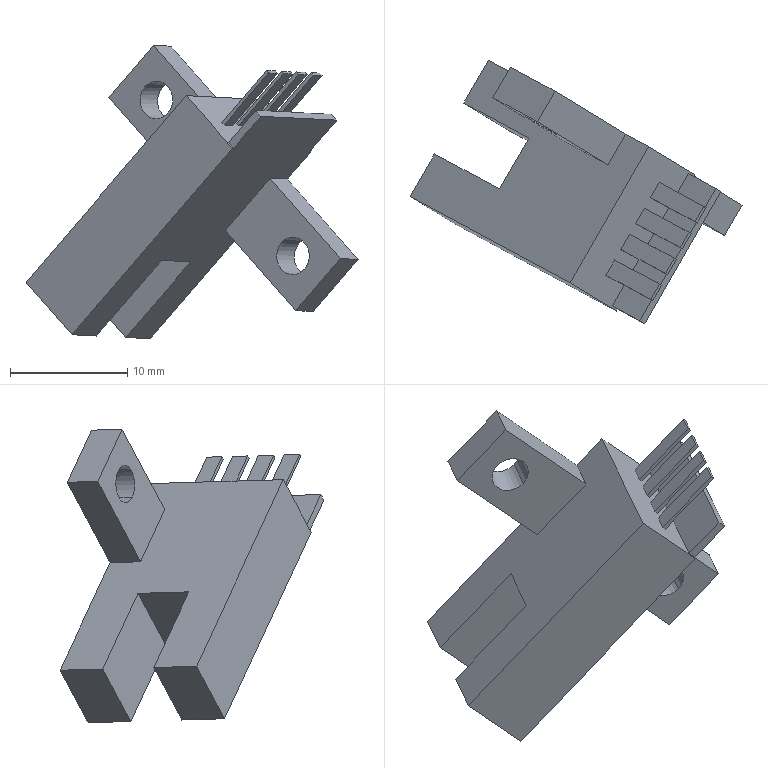Component | SolidWorks | KKSwitch-0710z0-123-1_EE-SX672-0710z0-123-4 | 1 solid | 46 faces | box 28.26 x 22.46 x 24.98 mm | volume 1978 mm3 | plane 42 | cylinder 4 | commonest cylinder face diameters 3.2 x4
build123d program:
from build123d import *

# Parameters (mm, degrees)
SKETCH1_W           = 13.4
SKETCH1_H           = 22.2
BOSS_EXTRUDE1_DEPTH = 6.4
SKETCH2_W           = 5
SKETCH2_H           = 9
CUT_EXTRUDE1_DEPTH  = 27.709
SKETCH3_W           = 1.5
SKETCH3_H           = 0.3
BOSS_EXTRUDE2_DEPTH = 6.2
SKETCH4_W           = 1.5
SKETCH4_H           = 0.3
BOSS_EXTRUDE3_DEPTH = 6.2
SKETCH5_W           = 1.5
SKETCH5_H           = 0.3
BOSS_EXTRUDE4_DEPTH = 6.2
SKETCH6_W           = 3
SKETCH6_H           = 6.2
BOSS_EXTRUDE5_DEPTH = 9.8
SKETCH7_W           = 3
SKETCH7_H           = 6.2
BOSS_EXTRUDE6_DEPTH = 9.8
SKETCH8_W           = 13
SKETCH8_H           = 0.7
BOSS_EXTRUDE7_DEPTH = 3.8
SKETCH9_W           = 1.5
SKETCH9_H           = 0.3
BOSS_EXTRUDE8_DEPTH = 6.2
DRILL1_D            = 3.2
DRILL2_D            = 3.2


with BuildPart() as part:
    # Sketch1 → Boss-Extrude1 (new body)
    with BuildSketch(Plane(origin=(0, 0, 0), x_dir=(-1, 0, 0), z_dir=(0, 0, -1))):
        with Locations((-6.7, 11.1)):
            Rectangle(SKETCH1_W, SKETCH1_H)
    extrude(amount=-BOSS_EXTRUDE1_DEPTH)

    # Sketch2 → Cut-Extrude1 (cut, through all)
    with BuildSketch(Plane(origin=(0, 0, 0), x_dir=(-1, 0, 0), z_dir=(0, 0, -1))):
        with Locations((-6.7, 17.7)):
            Rectangle(SKETCH2_W, SKETCH2_H)
    extrude(amount=-CUT_EXTRUDE1_DEPTH, mode=Mode.SUBTRACT)

    # Sketch3 → Boss-Extrude2 (add)
    with BuildSketch(Plane.XZ):
        with Locations((10.51, 3.05)):
            Rectangle(SKETCH3_W, SKETCH3_H)
    extrude(amount=BOSS_EXTRUDE2_DEPTH)

    # Sketch4 → Boss-Extrude3 (add)
    with BuildSketch(Plane.XZ):
        with Locations((5.43, 3.05)):
            Rectangle(SKETCH4_W, SKETCH4_H)
    extrude(amount=BOSS_EXTRUDE3_DEPTH)

    # Sketch5 → Boss-Extrude4 (add)
    with BuildSketch(Plane.XZ):
        with Locations((7.97, 3.05)):
            Rectangle(SKETCH5_W, SKETCH5_H)
    extrude(amount=BOSS_EXTRUDE4_DEPTH)

    # Sketch6 → Boss-Extrude5 (add)
    with BuildSketch(Plane.XY.offset(6.4)):
        with Locations((11.9, 6.3)):
            Rectangle(SKETCH6_W, SKETCH6_H)
    extrude(amount=BOSS_EXTRUDE5_DEPTH)

    # Sketch7 → Boss-Extrude6 (add)
    with BuildSketch(Plane(origin=(0, 0, 0), x_dir=(-1, 0, 0), z_dir=(0, 0, -1))):
        with Locations((-11.9, 6.3)):
            Rectangle(SKETCH7_W, SKETCH7_H)
    extrude(amount=BOSS_EXTRUDE6_DEPTH)

    # Sketch8 → Boss-Extrude7 (add)
    with BuildSketch(Plane.XZ):
        with Locations((6.7, 0.35)):
            Rectangle(SKETCH8_W, SKETCH8_H)
    extrude(amount=BOSS_EXTRUDE7_DEPTH)

    # Sketch9 → Boss-Extrude8 (add)
    with BuildSketch(Plane.XZ):
        with Locations((2.89, 3.05)):
            Rectangle(SKETCH9_W, SKETCH9_H)
    extrude(amount=BOSS_EXTRUDE8_DEPTH)

    # Drill1 (through all)
    with Locations(Plane.ZY.offset(-10.4)):
        with Locations((12.7, 6.3)):
            Hole(DRILL1_D / 2)

    # Drill2 (through all)
    with Locations(Plane.ZY.offset(-10.4)):
        with Locations((-6.3, 6.3)):
            Hole(DRILL2_D / 2)


solid = part.part

# Placed as in the assembly
solid = solid.moved(Location((68.276, -27.312, 239.836), (-28.021, -37.728, 51.003)))